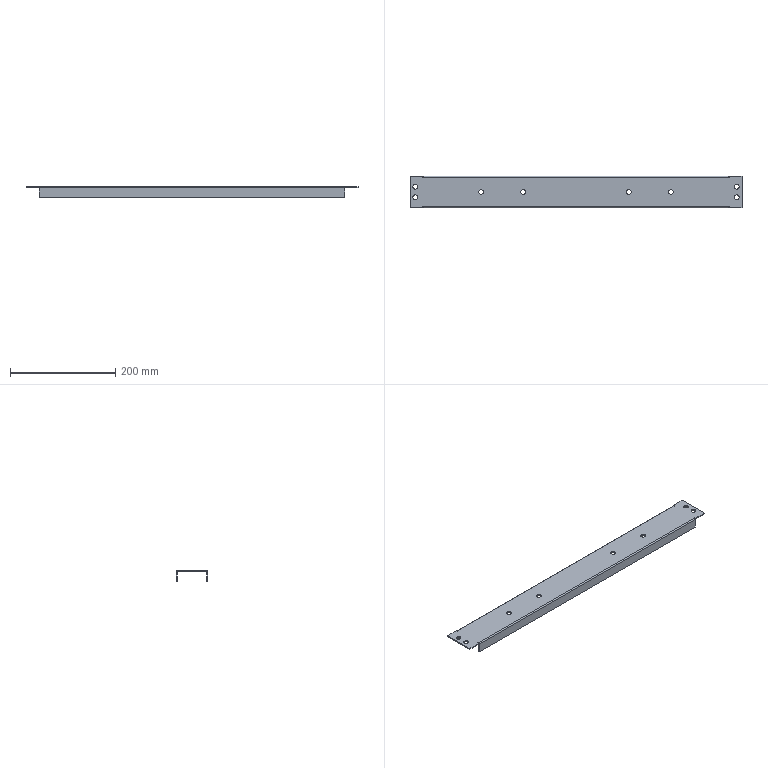Component | SolidWorks | KSHE-016.011-5 | 1 solid | 54 faces | volume 115222 mm3 | plane 34 | cylinder 20 | commonest cylinder face diameters 9 x16 4.2 x2 0.2 x2